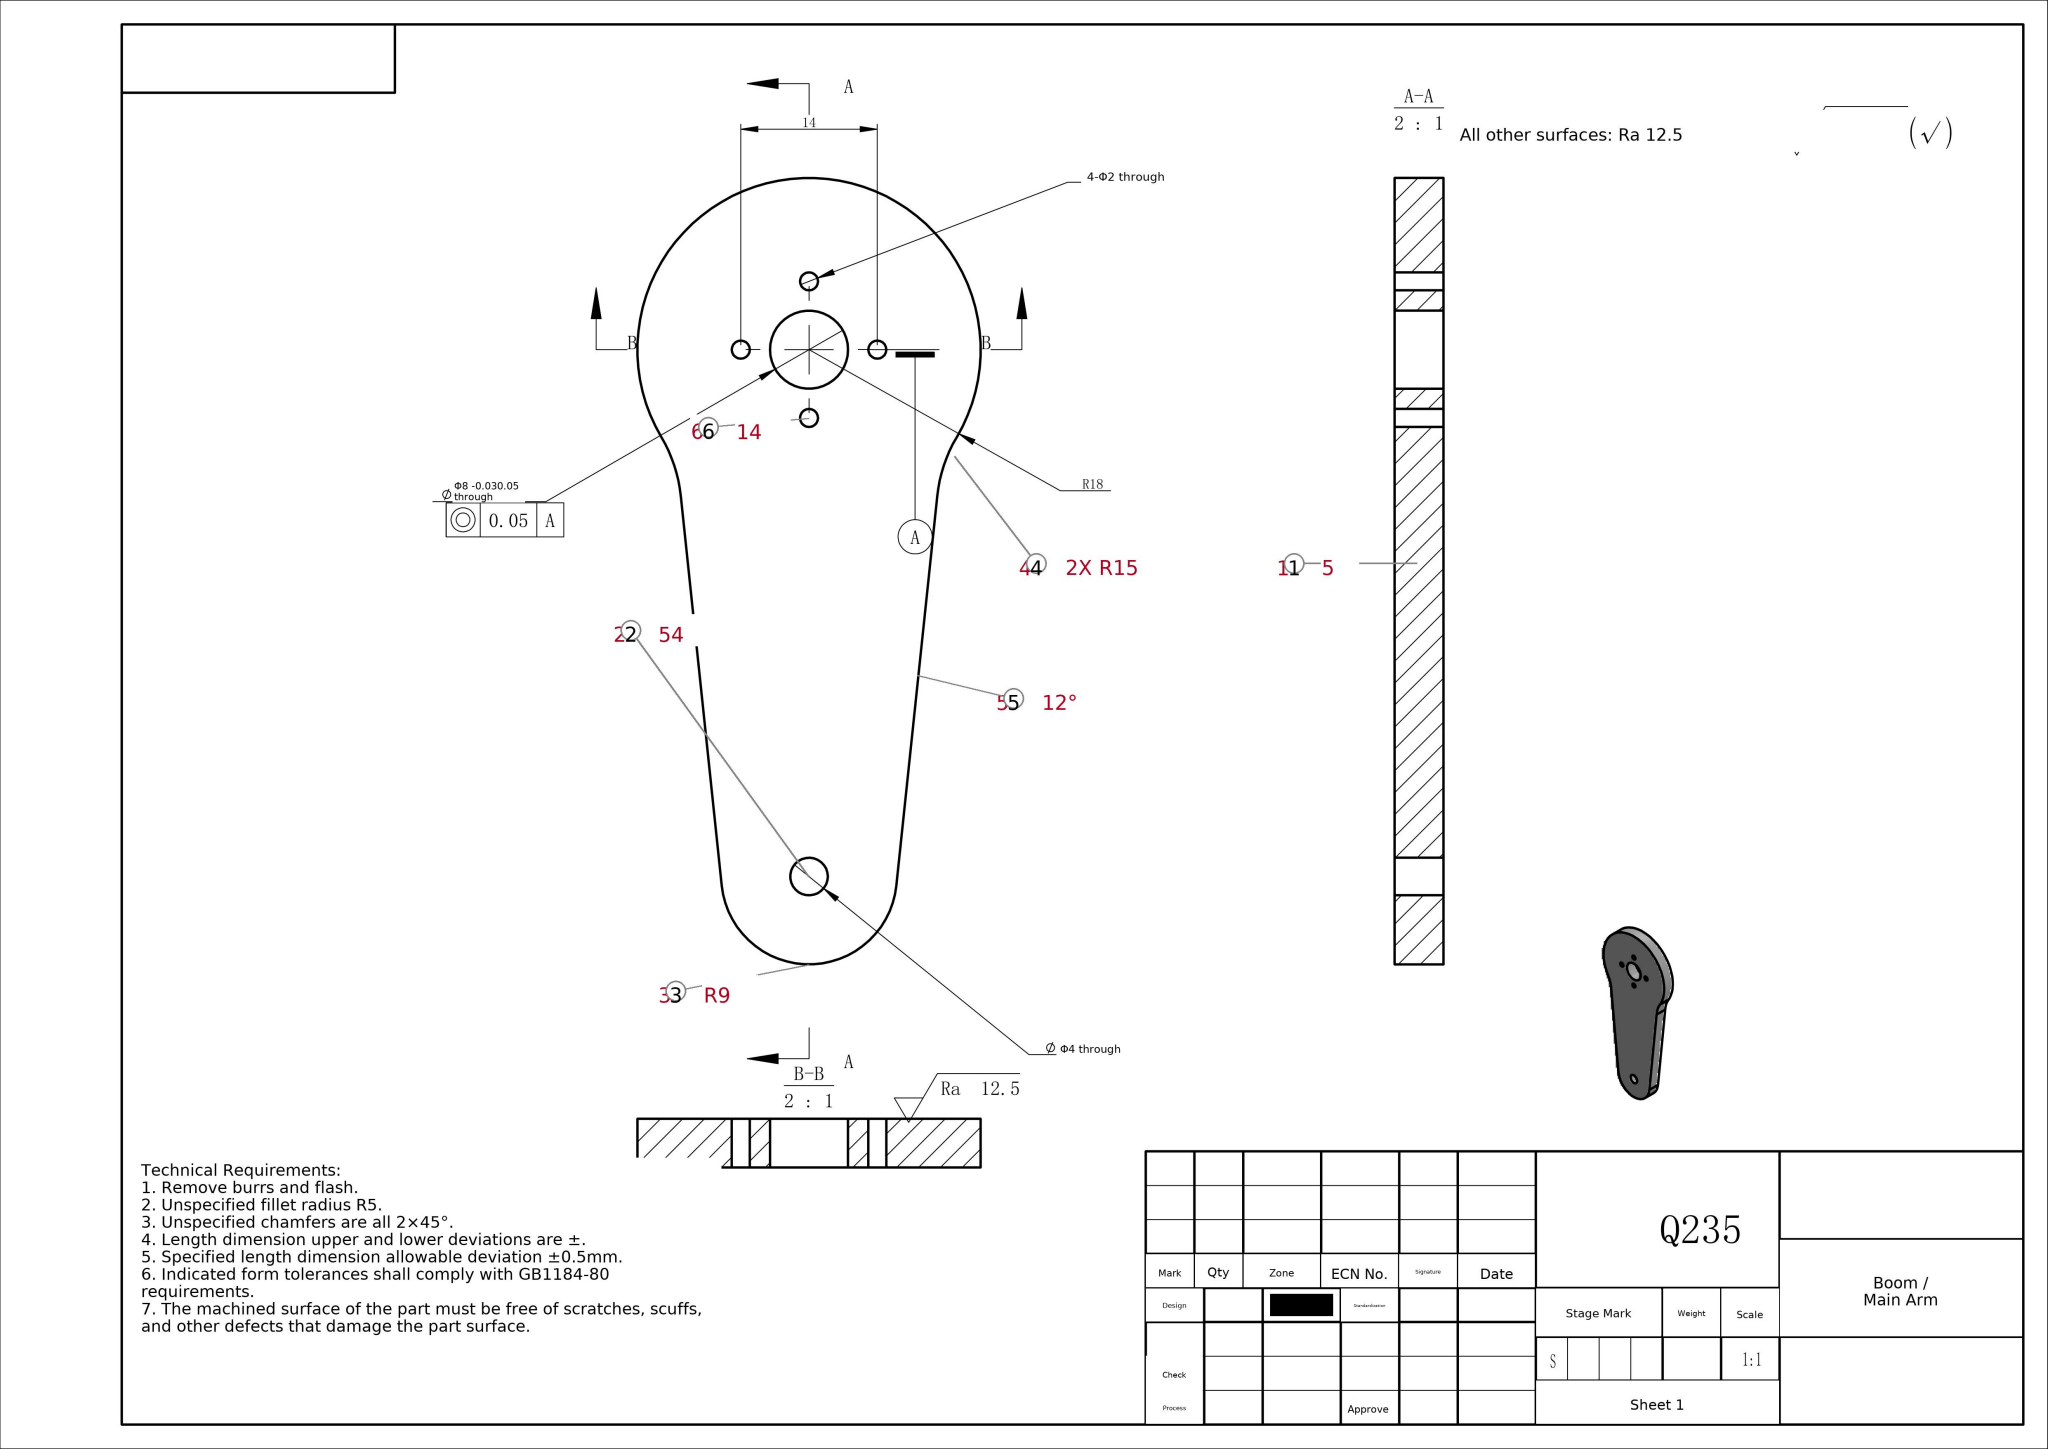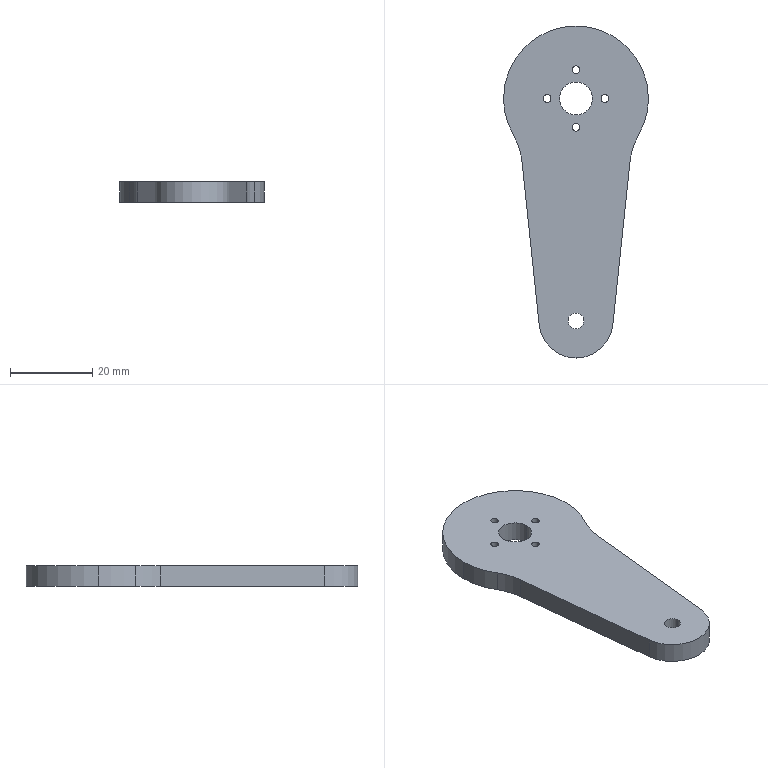Part | SolidWorks | mm | material Q235 | 1 solid | 22 faces | box 35.2 x 80.6 x 5 mm | volume 9381 mm3 | cylinder 18 | plane 4 | commonest cylinder face diameters 1.85 x8 35.2 x3 8 x2 3.85 x2 30 x2 18 x1
build123d program:
from build123d import *

# Parameters (mm, degrees)
ESQUISSE1_R        = 1.925
ESQUISSE1_R_2      = 0.925
ESQUISSE1_R_3      = 4
BOSS_EXTRU_1_DEPTH = 5


with BuildPart() as part:
    # Esquisse1 → Boss.-Extru.1 (new body)
    with BuildSketch(Plane.XY):
        with BuildLine():
            Line((8.951, -54.941), (13.147, -15.02))
            ThreePointArc((13.147, -15.02), (13.822, -11.88), (15.151, -8.955))
            ThreePointArc((15.151, -8.955), (0, 17.6), (-15.151, -8.955))
            ThreePointArc((-15.151, -8.955), (-13.822, -11.88), (-13.147, -15.02))
            Line((-13.147, -15.02), (-8.951, -54.941))
            ThreePointArc((-8.951, -54.941), (0, -63), (8.951, -54.941))
        make_face()
        with Locations((0, -54)):
            Circle(ESQUISSE1_R, mode=Mode.SUBTRACT)
        with Locations((7, 0)):
            Circle(ESQUISSE1_R_2, mode=Mode.SUBTRACT)
        with Locations((0, -7)):
            Circle(ESQUISSE1_R_2, mode=Mode.SUBTRACT)
        with Locations((0, 7)):
            Circle(ESQUISSE1_R_2, mode=Mode.SUBTRACT)
        with Locations((-7, 0)):
            Circle(ESQUISSE1_R_2, mode=Mode.SUBTRACT)
        Circle(ESQUISSE1_R_3, mode=Mode.SUBTRACT)
    extrude(amount=BOSS_EXTRU_1_DEPTH)


solid = part.part
STEP:
#1=CARTESIAN_POINT('',(-4.,0.,5.));
#2=VERTEX_POINT('',#1);
#3=CARTESIAN_POINT('',(4.,0.,5.));
#4=VERTEX_POINT('',#3);
#5=CARTESIAN_POINT('',(0.,0.,5.));
#6=DIRECTION('',(0.,0.,1.));
#7=DIRECTION('',(1.,0.,0.));
#8=AXIS2_PLACEMENT_3D('',#5,#6,#7);
#9=CIRCLE('',#8,4.);
#10=EDGE_CURVE('',#2,#4,#9,.T.);
#11=ORIENTED_EDGE('',*,*,#10,.T.);
#12=CARTESIAN_POINT('',(4.,0.,0.));
#13=VERTEX_POINT('',#12);
#14=CARTESIAN_POINT('',(4.,0.,5.));
#15=DIRECTION('',(0.,0.,-1.));
#16=VECTOR('',#15,1000.);
#17=LINE('',#14,#16);
#18=EDGE_CURVE('',#4,#13,#17,.T.);
#19=ORIENTED_EDGE('',*,*,#18,.T.);
#20=CARTESIAN_POINT('',(-4.,0.,0.));
#21=VERTEX_POINT('',#20);
#22=CARTESIAN_POINT('',(0.,0.,0.));
#23=DIRECTION('',(0.,0.,1.));
#24=DIRECTION('',(1.,0.,0.));
#25=AXIS2_PLACEMENT_3D('',#22,#23,#24);
#26=CIRCLE('',#25,4.);
#27=EDGE_CURVE('',#21,#13,#26,.T.);
#28=ORIENTED_EDGE('',*,*,#27,.F.);
#29=CARTESIAN_POINT('',(-4.,0.,5.));
#30=DIRECTION('',(0.,0.,-1.));
#31=VECTOR('',#30,1000.);
#32=LINE('',#29,#31);
#33=EDGE_CURVE('',#2,#21,#32,.T.);
#34=ORIENTED_EDGE('',*,*,#33,.F.);
#35=EDGE_LOOP('',(#11,#19,#28,#34));
#36=FACE_OUTER_BOUND('',#35,.T.);
#37=CARTESIAN_POINT('',(0.,0.,5.));
#38=DIRECTION('',(0.,0.,-1.));
#39=DIRECTION('',(-1.,0.,0.));
#40=AXIS2_PLACEMENT_3D('',#37,#38,#39);
#41=CYLINDRICAL_SURFACE('',#40,4.);
#42=ADVANCED_FACE('',(#36),#41,.F.);
#43=CARTESIAN_POINT('',(-7.925,0.,5.));
#44=VERTEX_POINT('',#43);
#45=CARTESIAN_POINT('',(-6.075,0.,5.));
#46=VERTEX_POINT('',#45);
#47=CARTESIAN_POINT('',(-7.,0.,5.));
#48=DIRECTION('',(0.,0.,1.));
#49=DIRECTION('',(1.,0.,0.));
#50=AXIS2_PLACEMENT_3D('',#47,#48,#49);
#51=CIRCLE('',#50,0.925);
#52=EDGE_CURVE('',#44,#46,#51,.T.);
#53=ORIENTED_EDGE('',*,*,#52,.T.);
#54=CARTESIAN_POINT('',(-6.075,0.,0.));
#55=VERTEX_POINT('',#54);
#56=CARTESIAN_POINT('',(-6.075,0.,5.));
#57=DIRECTION('',(0.,0.,-1.));
#58=VECTOR('',#57,1000.);
#59=LINE('',#56,#58);
#60=EDGE_CURVE('',#46,#55,#59,.T.);
#61=ORIENTED_EDGE('',*,*,#60,.T.);
#62=CARTESIAN_POINT('',(-7.925,0.,0.));
#63=VERTEX_POINT('',#62);
#64=CARTESIAN_POINT('',(-7.,0.,0.));
#65=DIRECTION('',(0.,0.,1.));
#66=DIRECTION('',(1.,0.,0.));
#67=AXIS2_PLACEMENT_3D('',#64,#65,#66);
#68=CIRCLE('',#67,0.925);
#69=EDGE_CURVE('',#63,#55,#68,.T.);
#70=ORIENTED_EDGE('',*,*,#69,.F.);
#71=CARTESIAN_POINT('',(-7.925,0.,5.));
#72=DIRECTION('',(0.,0.,-1.));
#73=VECTOR('',#72,1000.);
#74=LINE('',#71,#73);
#75=EDGE_CURVE('',#44,#63,#74,.T.);
#76=ORIENTED_EDGE('',*,*,#75,.F.);
#77=EDGE_LOOP('',(#53,#61,#70,#76));
#78=FACE_OUTER_BOUND('',#77,.T.);
#79=CARTESIAN_POINT('',(-7.,0.,5.));
#80=DIRECTION('',(0.,0.,-1.));
#81=DIRECTION('',(-1.,0.,0.));
#82=AXIS2_PLACEMENT_3D('',#79,#80,#81);
#83=CYLINDRICAL_SURFACE('',#82,0.925);
#84=ADVANCED_FACE('',(#78),#83,.F.);
#85=CARTESIAN_POINT('',(-0.925,7.,5.));
#86=VERTEX_POINT('',#85);
#87=CARTESIAN_POINT('',(0.925,7.,5.));
#88=VERTEX_POINT('',#87);
#89=CARTESIAN_POINT('',(0.,7.,5.));
#90=DIRECTION('',(0.,0.,1.));
#91=DIRECTION('',(1.,0.,0.));
#92=AXIS2_PLACEMENT_3D('',#89,#90,#91);
#93=CIRCLE('',#92,0.925);
#94=EDGE_CURVE('',#86,#88,#93,.T.);
#95=ORIENTED_EDGE('',*,*,#94,.T.);
#96=CARTESIAN_POINT('',(0.925,7.,0.));
#97=VERTEX_POINT('',#96);
#98=CARTESIAN_POINT('',(0.925,7.,5.));
#99=DIRECTION('',(0.,0.,-1.));
#100=VECTOR('',#99,1000.);
#101=LINE('',#98,#100);
#102=EDGE_CURVE('',#88,#97,#101,.T.);
#103=ORIENTED_EDGE('',*,*,#102,.T.);
#104=CARTESIAN_POINT('',(-0.925,7.,0.));
#105=VERTEX_POINT('',#104);
#106=CARTESIAN_POINT('',(0.,7.,0.));
#107=DIRECTION('',(0.,0.,1.));
#108=DIRECTION('',(1.,0.,0.));
#109=AXIS2_PLACEMENT_3D('',#106,#107,#108);
#110=CIRCLE('',#109,0.925);
#111=EDGE_CURVE('',#105,#97,#110,.T.);
#112=ORIENTED_EDGE('',*,*,#111,.F.);
#113=CARTESIAN_POINT('',(-0.925,7.,5.));
#114=DIRECTION('',(0.,0.,-1.));
#115=VECTOR('',#114,1000.);
#116=LINE('',#113,#115);
#117=EDGE_CURVE('',#86,#105,#116,.T.);
#118=ORIENTED_EDGE('',*,*,#117,.F.);
#119=EDGE_LOOP('',(#95,#103,#112,#118));
#120=FACE_OUTER_BOUND('',#119,.T.);
#121=CARTESIAN_POINT('',(0.,7.,5.));
#122=DIRECTION('',(0.,0.,-1.));
#123=DIRECTION('',(-1.,0.,0.));
#124=AXIS2_PLACEMENT_3D('',#121,#122,#123);
#125=CYLINDRICAL_SURFACE('',#124,0.925);
#126=ADVANCED_FACE('',(#120),#125,.F.);
#127=CARTESIAN_POINT('',(-0.925,-7.,5.));
#128=VERTEX_POINT('',#127);
#129=CARTESIAN_POINT('',(0.925,-7.,5.));
#130=VERTEX_POINT('',#129);
#131=CARTESIAN_POINT('',(0.,-7.,5.));
#132=DIRECTION('',(0.,0.,1.));
#133=DIRECTION('',(1.,0.,0.));
#134=AXIS2_PLACEMENT_3D('',#131,#132,#133);
#135=CIRCLE('',#134,0.925);
#136=EDGE_CURVE('',#128,#130,#135,.T.);
#137=ORIENTED_EDGE('',*,*,#136,.T.);
#138=CARTESIAN_POINT('',(0.925,-7.,0.));
#139=VERTEX_POINT('',#138);
#140=CARTESIAN_POINT('',(0.925,-7.,5.));
#141=DIRECTION('',(0.,0.,-1.));
#142=VECTOR('',#141,1000.);
#143=LINE('',#140,#142);
#144=EDGE_CURVE('',#130,#139,#143,.T.);
#145=ORIENTED_EDGE('',*,*,#144,.T.);
#146=CARTESIAN_POINT('',(-0.925,-7.,0.));
#147=VERTEX_POINT('',#146);
#148=CARTESIAN_POINT('',(0.,-7.,0.));
#149=DIRECTION('',(0.,0.,1.));
#150=DIRECTION('',(1.,0.,0.));
#151=AXIS2_PLACEMENT_3D('',#148,#149,#150);
#152=CIRCLE('',#151,0.925);
#153=EDGE_CURVE('',#147,#139,#152,.T.);
#154=ORIENTED_EDGE('',*,*,#153,.F.);
#155=CARTESIAN_POINT('',(-0.925,-7.,5.));
#156=DIRECTION('',(0.,0.,-1.));
#157=VECTOR('',#156,1000.);
#158=LINE('',#155,#157);
#159=EDGE_CURVE('',#128,#147,#158,.T.);
#160=ORIENTED_EDGE('',*,*,#159,.F.);
#161=EDGE_LOOP('',(#137,#145,#154,#160));
#162=FACE_OUTER_BOUND('',#161,.T.);
#163=CARTESIAN_POINT('',(0.,-7.,5.));
#164=DIRECTION('',(0.,0.,-1.));
#165=DIRECTION('',(-1.,0.,0.));
#166=AXIS2_PLACEMENT_3D('',#163,#164,#165);
#167=CYLINDRICAL_SURFACE('',#166,0.925);
#168=ADVANCED_FACE('',(#162),#167,.F.);
#169=CARTESIAN_POINT('',(6.075,0.,5.));
#170=VERTEX_POINT('',#169);
#171=CARTESIAN_POINT('',(7.925,0.,5.));
#172=VERTEX_POINT('',#171);
#173=CARTESIAN_POINT('',(7.,0.,5.));
#174=DIRECTION('',(0.,0.,1.));
#175=DIRECTION('',(1.,0.,0.));
#176=AXIS2_PLACEMENT_3D('',#173,#174,#175);
#177=CIRCLE('',#176,0.925);
#178=EDGE_CURVE('',#170,#172,#177,.T.);
#179=ORIENTED_EDGE('',*,*,#178,.T.);
#180=CARTESIAN_POINT('',(7.925,0.,0.));
#181=VERTEX_POINT('',#180);
#182=CARTESIAN_POINT('',(7.925,0.,5.));
#183=DIRECTION('',(0.,0.,-1.));
#184=VECTOR('',#183,1000.);
#185=LINE('',#182,#184);
#186=EDGE_CURVE('',#172,#181,#185,.T.);
#187=ORIENTED_EDGE('',*,*,#186,.T.);
#188=CARTESIAN_POINT('',(6.075,0.,0.));
#189=VERTEX_POINT('',#188);
#190=CARTESIAN_POINT('',(7.,0.,0.));
#191=DIRECTION('',(0.,0.,1.));
#192=DIRECTION('',(1.,0.,0.));
#193=AXIS2_PLACEMENT_3D('',#190,#191,#192);
#194=CIRCLE('',#193,0.925);
#195=EDGE_CURVE('',#189,#181,#194,.T.);
#196=ORIENTED_EDGE('',*,*,#195,.F.);
#197=CARTESIAN_POINT('',(6.075,0.,5.));
#198=DIRECTION('',(0.,0.,-1.));
#199=VECTOR('',#198,1000.);
#200=LINE('',#197,#199);
#201=EDGE_CURVE('',#170,#189,#200,.T.);
#202=ORIENTED_EDGE('',*,*,#201,.F.);
#203=EDGE_LOOP('',(#179,#187,#196,#202));
#204=FACE_OUTER_BOUND('',#203,.T.);
#205=CARTESIAN_POINT('',(7.,0.,5.));
#206=DIRECTION('',(0.,0.,-1.));
#207=DIRECTION('',(-1.,0.,0.));
#208=AXIS2_PLACEMENT_3D('',#205,#206,#207);
#209=CYLINDRICAL_SURFACE('',#208,0.925);
#210=ADVANCED_FACE('',(#204),#209,.F.);
#211=CARTESIAN_POINT('',(-1.925,-54.,5.));
#212=VERTEX_POINT('',#211);
#213=CARTESIAN_POINT('',(1.925,-54.,5.));
#214=VERTEX_POINT('',#213);
#215=CARTESIAN_POINT('',(0.,-54.,5.));
#216=DIRECTION('',(0.,0.,1.));
#217=DIRECTION('',(1.,0.,0.));
#218=AXIS2_PLACEMENT_3D('',#215,#216,#217);
#219=CIRCLE('',#218,1.925);
#220=EDGE_CURVE('',#212,#214,#219,.T.);
#221=ORIENTED_EDGE('',*,*,#220,.T.);
#222=CARTESIAN_POINT('',(1.925,-54.,0.));
#223=VERTEX_POINT('',#222);
#224=CARTESIAN_POINT('',(1.925,-54.,5.));
#225=DIRECTION('',(0.,0.,-1.));
#226=VECTOR('',#225,1000.);
#227=LINE('',#224,#226);
#228=EDGE_CURVE('',#214,#223,#227,.T.);
#229=ORIENTED_EDGE('',*,*,#228,.T.);
#230=CARTESIAN_POINT('',(-1.925,-54.,0.));
#231=VERTEX_POINT('',#230);
#232=CARTESIAN_POINT('',(0.,-54.,0.));
#233=DIRECTION('',(0.,0.,1.));
#234=DIRECTION('',(1.,0.,0.));
#235=AXIS2_PLACEMENT_3D('',#232,#233,#234);
#236=CIRCLE('',#235,1.925);
#237=EDGE_CURVE('',#231,#223,#236,.T.);
#238=ORIENTED_EDGE('',*,*,#237,.F.);
#239=CARTESIAN_POINT('',(-1.925,-54.,5.));
#240=DIRECTION('',(0.,0.,-1.));
#241=VECTOR('',#240,1000.);
#242=LINE('',#239,#241);
#243=EDGE_CURVE('',#212,#231,#242,.T.);
#244=ORIENTED_EDGE('',*,*,#243,.F.);
#245=EDGE_LOOP('',(#221,#229,#238,#244));
#246=FACE_OUTER_BOUND('',#245,.T.);
#247=CARTESIAN_POINT('',(0.,-54.,5.));
#248=DIRECTION('',(0.,0.,-1.));
#249=DIRECTION('',(-1.,0.,0.));
#250=AXIS2_PLACEMENT_3D('',#247,#248,#249);
#251=CYLINDRICAL_SURFACE('',#250,1.925);
#252=ADVANCED_FACE('',(#246),#251,.F.);
#253=CARTESIAN_POINT('',(17.6,0.,5.));
#254=VERTEX_POINT('',#253);
#255=CARTESIAN_POINT('',(-17.6,0.,5.));
#256=VERTEX_POINT('',#255);
#257=CARTESIAN_POINT('',(0.,0.,5.));
#258=DIRECTION('',(0.,0.,1.));
#259=DIRECTION('',(1.,0.,0.));
#260=AXIS2_PLACEMENT_3D('',#257,#258,#259);
#261=CIRCLE('',#260,17.6);
#262=EDGE_CURVE('',#254,#256,#261,.T.);
#263=ORIENTED_EDGE('',*,*,#262,.F.);
#264=CARTESIAN_POINT('',(17.6,0.,0.));
#265=VERTEX_POINT('',#264);
#266=CARTESIAN_POINT('',(17.6,0.,5.));
#267=DIRECTION('',(0.,0.,-1.));
#268=VECTOR('',#267,1000.);
#269=LINE('',#266,#268);
#270=EDGE_CURVE('',#254,#265,#269,.T.);
#271=ORIENTED_EDGE('',*,*,#270,.T.);
#272=CARTESIAN_POINT('',(-17.6,0.,0.));
#273=VERTEX_POINT('',#272);
#274=CARTESIAN_POINT('',(0.,0.,0.));
#275=DIRECTION('',(0.,0.,1.));
#276=DIRECTION('',(1.,0.,0.));
#277=AXIS2_PLACEMENT_3D('',#274,#275,#276);
#278=CIRCLE('',#277,17.6);
#279=EDGE_CURVE('',#265,#273,#278,.T.);
#280=ORIENTED_EDGE('',*,*,#279,.T.);
#281=CARTESIAN_POINT('',(-17.6,0.,5.));
#282=DIRECTION('',(0.,0.,-1.));
#283=VECTOR('',#282,1000.);
#284=LINE('',#281,#283);
#285=EDGE_CURVE('',#256,#273,#284,.T.);
#286=ORIENTED_EDGE('',*,*,#285,.F.);
#287=EDGE_LOOP('',(#263,#271,#280,#286));
#288=FACE_OUTER_BOUND('',#287,.T.);
#289=CARTESIAN_POINT('',(0.,0.,5.));
#290=DIRECTION('',(0.,0.,-1.));
#291=DIRECTION('',(-1.,0.,0.));
#292=AXIS2_PLACEMENT_3D('',#289,#290,#291);
#293=CYLINDRICAL_SURFACE('',#292,17.6);
#294=ADVANCED_FACE('',(#288),#293,.T.);
#295=CARTESIAN_POINT('',(-15.151,-8.955,5.));
#296=VERTEX_POINT('',#295);
#297=CARTESIAN_POINT('',(0.,0.,5.));
#298=DIRECTION('',(0.,0.,1.));
#299=DIRECTION('',(1.,0.,0.));
#300=AXIS2_PLACEMENT_3D('',#297,#298,#299);
#301=CIRCLE('',#300,17.6);
#302=EDGE_CURVE('',#256,#296,#301,.T.);
#303=ORIENTED_EDGE('',*,*,#302,.F.);
#304=ORIENTED_EDGE('',*,*,#285,.T.);
#305=CARTESIAN_POINT('',(-15.151,-8.955,0.));
#306=VERTEX_POINT('',#305);
#307=CARTESIAN_POINT('',(0.,0.,0.));
#308=DIRECTION('',(0.,0.,1.));
#309=DIRECTION('',(1.,0.,0.));
#310=AXIS2_PLACEMENT_3D('',#307,#308,#309);
#311=CIRCLE('',#310,17.6);
#312=EDGE_CURVE('',#273,#306,#311,.T.);
#313=ORIENTED_EDGE('',*,*,#312,.T.);
#314=CARTESIAN_POINT('',(-15.151,-8.955,5.));
#315=DIRECTION('',(0.,0.,-1.));
#316=VECTOR('',#315,1000.);
#317=LINE('',#314,#316);
#318=EDGE_CURVE('',#296,#306,#317,.T.);
#319=ORIENTED_EDGE('',*,*,#318,.F.);
#320=EDGE_LOOP('',(#303,#304,#313,#319));
#321=FACE_OUTER_BOUND('',#320,.T.);
#322=CARTESIAN_POINT('',(0.,0.,5.));
#323=DIRECTION('',(0.,0.,-1.));
#324=DIRECTION('',(-1.,0.,0.));
#325=AXIS2_PLACEMENT_3D('',#322,#323,#324);
#326=CYLINDRICAL_SURFACE('',#325,17.6);
#327=ADVANCED_FACE('',(#321),#326,.T.);
#328=ORIENTED_EDGE('',*,*,#52,.F.);
#329=CARTESIAN_POINT('',(-7.,0.,5.));
#330=DIRECTION('',(0.,0.,1.));
#331=DIRECTION('',(1.,0.,0.));
#332=AXIS2_PLACEMENT_3D('',#329,#330,#331);
#333=CIRCLE('',#332,0.925);
#334=EDGE_CURVE('',#46,#44,#333,.T.);
#335=ORIENTED_EDGE('',*,*,#334,.F.);
#336=EDGE_LOOP('',(#328,#335));
#337=FACE_BOUND('',#336,.T.);
#338=ORIENTED_EDGE('',*,*,#136,.F.);
#339=CARTESIAN_POINT('',(0.,-7.,5.));
#340=DIRECTION('',(0.,0.,1.));
#341=DIRECTION('',(1.,0.,0.));
#342=AXIS2_PLACEMENT_3D('',#339,#340,#341);
#343=CIRCLE('',#342,0.925);
#344=EDGE_CURVE('',#130,#128,#343,.T.);
#345=ORIENTED_EDGE('',*,*,#344,.F.);
#346=EDGE_LOOP('',(#338,#345));
#347=FACE_BOUND('',#346,.T.);
#348=ORIENTED_EDGE('',*,*,#220,.F.);
#349=CARTESIAN_POINT('',(0.,-54.,5.));
#350=DIRECTION('',(0.,0.,1.));
#351=DIRECTION('',(1.,0.,0.));
#352=AXIS2_PLACEMENT_3D('',#349,#350,#351);
#353=CIRCLE('',#352,1.925);
#354=EDGE_CURVE('',#214,#212,#353,.T.);
#355=ORIENTED_EDGE('',*,*,#354,.F.);
#356=EDGE_LOOP('',(#348,#355));
#357=FACE_BOUND('',#356,.T.);
#358=CARTESIAN_POINT('',(-8.951,-54.941,5.));
#359=VERTEX_POINT('',#358);
#360=CARTESIAN_POINT('',(8.951,-54.941,5.));
#361=VERTEX_POINT('',#360);
#362=CARTESIAN_POINT('',(0.,-54.,5.));
#363=DIRECTION('',(0.,0.,1.));
#364=DIRECTION('',(1.,0.,0.));
#365=AXIS2_PLACEMENT_3D('',#362,#363,#364);
#366=CIRCLE('',#365,9.);
#367=EDGE_CURVE('',#359,#361,#366,.T.);
#368=ORIENTED_EDGE('',*,*,#367,.T.);
#369=CARTESIAN_POINT('',(13.147,-15.02,5.));
#370=VERTEX_POINT('',#369);
#371=CARTESIAN_POINT('',(8.951,-54.941,5.));
#372=DIRECTION('',(0.1045,0.9945,0.));
#373=VECTOR('',#372,1000.);
#374=LINE('',#371,#373);
#375=EDGE_CURVE('',#361,#370,#374,.T.);
#376=ORIENTED_EDGE('',*,*,#375,.T.);
#377=CARTESIAN_POINT('',(15.151,-8.955,5.));
#378=VERTEX_POINT('',#377);
#379=CARTESIAN_POINT('',(28.064,-16.588,5.));
#380=DIRECTION('',(0.,0.,-1.));
#381=DIRECTION('',(1.,0.,0.));
#382=AXIS2_PLACEMENT_3D('',#379,#380,#381);
#383=CIRCLE('',#382,15.);
#384=EDGE_CURVE('',#370,#378,#383,.T.);
#385=ORIENTED_EDGE('',*,*,#384,.T.);
#386=CARTESIAN_POINT('',(0.,0.,5.));
#387=DIRECTION('',(0.,0.,1.));
#388=DIRECTION('',(1.,0.,0.));
#389=AXIS2_PLACEMENT_3D('',#386,#387,#388);
#390=CIRCLE('',#389,17.6);
#391=EDGE_CURVE('',#378,#254,#390,.T.);
#392=ORIENTED_EDGE('',*,*,#391,.T.);
#393=ORIENTED_EDGE('',*,*,#262,.T.);
#394=ORIENTED_EDGE('',*,*,#302,.T.);
#395=CARTESIAN_POINT('',(-13.147,-15.02,5.));
#396=VERTEX_POINT('',#395);
#397=CARTESIAN_POINT('',(-28.064,-16.588,5.));
#398=DIRECTION('',(0.,0.,-1.));
#399=DIRECTION('',(1.,0.,0.));
#400=AXIS2_PLACEMENT_3D('',#397,#398,#399);
#401=CIRCLE('',#400,15.);
#402=EDGE_CURVE('',#296,#396,#401,.T.);
#403=ORIENTED_EDGE('',*,*,#402,.T.);
#404=CARTESIAN_POINT('',(-13.147,-15.02,5.));
#405=DIRECTION('',(0.1045,-0.9945,0.));
#406=VECTOR('',#405,1000.);
#407=LINE('',#404,#406);
#408=EDGE_CURVE('',#396,#359,#407,.T.);
#409=ORIENTED_EDGE('',*,*,#408,.T.);
#410=EDGE_LOOP('',(#368,#376,#385,#392,#393,#394,#403,#409));
#411=FACE_OUTER_BOUND('',#410,.T.);
#412=ORIENTED_EDGE('',*,*,#178,.F.);
#413=CARTESIAN_POINT('',(7.,0.,5.));
#414=DIRECTION('',(0.,0.,1.));
#415=DIRECTION('',(1.,0.,0.));
#416=AXIS2_PLACEMENT_3D('',#413,#414,#415);
#417=CIRCLE('',#416,0.925);
#418=EDGE_CURVE('',#172,#170,#417,.T.);
#419=ORIENTED_EDGE('',*,*,#418,.F.);
#420=EDGE_LOOP('',(#412,#419));
#421=FACE_BOUND('',#420,.T.);
#422=ORIENTED_EDGE('',*,*,#94,.F.);
#423=CARTESIAN_POINT('',(0.,7.,5.));
#424=DIRECTION('',(0.,0.,1.));
#425=DIRECTION('',(1.,0.,0.));
#426=AXIS2_PLACEMENT_3D('',#423,#424,#425);
#427=CIRCLE('',#426,0.925);
#428=EDGE_CURVE('',#88,#86,#427,.T.);
#429=ORIENTED_EDGE('',*,*,#428,.F.);
#430=EDGE_LOOP('',(#422,#429));
#431=FACE_BOUND('',#430,.T.);
#432=ORIENTED_EDGE('',*,*,#10,.F.);
#433=CARTESIAN_POINT('',(0.,0.,5.));
#434=DIRECTION('',(0.,0.,1.));
#435=DIRECTION('',(1.,0.,0.));
#436=AXIS2_PLACEMENT_3D('',#433,#434,#435);
#437=CIRCLE('',#436,4.);
#438=EDGE_CURVE('',#4,#2,#437,.T.);
#439=ORIENTED_EDGE('',*,*,#438,.F.);
#440=EDGE_LOOP('',(#432,#439));
#441=FACE_BOUND('',#440,.T.);
#442=CARTESIAN_POINT('',(0.,-54.,5.));
#443=DIRECTION('',(0.,0.,1.));
#444=DIRECTION('',(1.,0.,0.));
#445=AXIS2_PLACEMENT_3D('',#442,#443,#444);
#446=PLANE('',#445);
#447=ADVANCED_FACE('',(#337,#347,#357,#411,#421,#431,#441),#446,.T.);
#448=CARTESIAN_POINT('',(-8.951,-54.941,0.));
#449=VERTEX_POINT('',#448);
#450=CARTESIAN_POINT('',(8.951,-54.941,0.));
#451=VERTEX_POINT('',#450);
#452=CARTESIAN_POINT('',(0.,-54.,0.));
#453=DIRECTION('',(0.,0.,1.));
#454=DIRECTION('',(1.,0.,0.));
#455=AXIS2_PLACEMENT_3D('',#452,#453,#454);
#456=CIRCLE('',#455,9.);
#457=EDGE_CURVE('',#449,#451,#456,.T.);
#458=ORIENTED_EDGE('',*,*,#457,.F.);
#459=CARTESIAN_POINT('',(-13.147,-15.02,0.));
#460=VERTEX_POINT('',#459);
#461=CARTESIAN_POINT('',(-13.147,-15.02,0.));
#462=DIRECTION('',(0.1045,-0.9945,0.));
#463=VECTOR('',#462,1000.);
#464=LINE('',#461,#463);
#465=EDGE_CURVE('',#460,#449,#464,.T.);
#466=ORIENTED_EDGE('',*,*,#465,.F.);
#467=CARTESIAN_POINT('',(-28.064,-16.588,0.));
#468=DIRECTION('',(0.,0.,-1.));
#469=DIRECTION('',(1.,0.,0.));
#470=AXIS2_PLACEMENT_3D('',#467,#468,#469);
#471=CIRCLE('',#470,15.);
#472=EDGE_CURVE('',#306,#460,#471,.T.);
#473=ORIENTED_EDGE('',*,*,#472,.F.);
#474=ORIENTED_EDGE('',*,*,#312,.F.);
#475=ORIENTED_EDGE('',*,*,#279,.F.);
#476=CARTESIAN_POINT('',(15.151,-8.955,0.));
#477=VERTEX_POINT('',#476);
#478=CARTESIAN_POINT('',(0.,0.,0.));
#479=DIRECTION('',(0.,0.,1.));
#480=DIRECTION('',(1.,0.,0.));
#481=AXIS2_PLACEMENT_3D('',#478,#479,#480);
#482=CIRCLE('',#481,17.6);
#483=EDGE_CURVE('',#477,#265,#482,.T.);
#484=ORIENTED_EDGE('',*,*,#483,.F.);
#485=CARTESIAN_POINT('',(13.147,-15.02,0.));
#486=VERTEX_POINT('',#485);
#487=CARTESIAN_POINT('',(28.064,-16.588,0.));
#488=DIRECTION('',(0.,0.,-1.));
#489=DIRECTION('',(1.,0.,0.));
#490=AXIS2_PLACEMENT_3D('',#487,#488,#489);
#491=CIRCLE('',#490,15.);
#492=EDGE_CURVE('',#486,#477,#491,.T.);
#493=ORIENTED_EDGE('',*,*,#492,.F.);
#494=CARTESIAN_POINT('',(8.951,-54.941,0.));
#495=DIRECTION('',(0.1045,0.9945,0.));
#496=VECTOR('',#495,1000.);
#497=LINE('',#494,#496);
#498=EDGE_CURVE('',#451,#486,#497,.T.);
#499=ORIENTED_EDGE('',*,*,#498,.F.);
#500=EDGE_LOOP('',(#458,#466,#473,#474,#475,#484,#493,#499));
#501=FACE_OUTER_BOUND('',#500,.T.);
#502=ORIENTED_EDGE('',*,*,#237,.T.);
#503=CARTESIAN_POINT('',(0.,-54.,0.));
#504=DIRECTION('',(0.,0.,1.));
#505=DIRECTION('',(1.,0.,0.));
#506=AXIS2_PLACEMENT_3D('',#503,#504,#505);
#507=CIRCLE('',#506,1.925);
#508=EDGE_CURVE('',#223,#231,#507,.T.);
#509=ORIENTED_EDGE('',*,*,#508,.T.);
#510=EDGE_LOOP('',(#502,#509));
#511=FACE_BOUND('',#510,.T.);
#512=ORIENTED_EDGE('',*,*,#195,.T.);
#513=CARTESIAN_POINT('',(7.,0.,0.));
#514=DIRECTION('',(0.,0.,1.));
#515=DIRECTION('',(1.,0.,0.));
#516=AXIS2_PLACEMENT_3D('',#513,#514,#515);
#517=CIRCLE('',#516,0.925);
#518=EDGE_CURVE('',#181,#189,#517,.T.);
#519=ORIENTED_EDGE('',*,*,#518,.T.);
#520=EDGE_LOOP('',(#512,#519));
#521=FACE_BOUND('',#520,.T.);
#522=ORIENTED_EDGE('',*,*,#153,.T.);
#523=CARTESIAN_POINT('',(0.,-7.,0.));
#524=DIRECTION('',(0.,0.,1.));
#525=DIRECTION('',(1.,0.,0.));
#526=AXIS2_PLACEMENT_3D('',#523,#524,#525);
#527=CIRCLE('',#526,0.925);
#528=EDGE_CURVE('',#139,#147,#527,.T.);
#529=ORIENTED_EDGE('',*,*,#528,.T.);
#530=EDGE_LOOP('',(#522,#529));
#531=FACE_BOUND('',#530,.T.);
#532=ORIENTED_EDGE('',*,*,#111,.T.);
#533=CARTESIAN_POINT('',(0.,7.,0.));
#534=DIRECTION('',(0.,0.,1.));
#535=DIRECTION('',(1.,0.,0.));
#536=AXIS2_PLACEMENT_3D('',#533,#534,#535);
#537=CIRCLE('',#536,0.925);
#538=EDGE_CURVE('',#97,#105,#537,.T.);
#539=ORIENTED_EDGE('',*,*,#538,.T.);
#540=EDGE_LOOP('',(#532,#539));
#541=FACE_BOUND('',#540,.T.);
#542=ORIENTED_EDGE('',*,*,#69,.T.);
#543=CARTESIAN_POINT('',(-7.,0.,0.));
#544=DIRECTION('',(0.,0.,1.));
#545=DIRECTION('',(1.,0.,0.));
#546=AXIS2_PLACEMENT_3D('',#543,#544,#545);
#547=CIRCLE('',#546,0.925);
#548=EDGE_CURVE('',#55,#63,#547,.T.);
#549=ORIENTED_EDGE('',*,*,#548,.T.);
#550=EDGE_LOOP('',(#542,#549));
#551=FACE_BOUND('',#550,.T.);
#552=ORIENTED_EDGE('',*,*,#27,.T.);
#553=CARTESIAN_POINT('',(0.,0.,0.));
#554=DIRECTION('',(0.,0.,1.));
#555=DIRECTION('',(1.,0.,0.));
#556=AXIS2_PLACEMENT_3D('',#553,#554,#555);
#557=CIRCLE('',#556,4.);
#558=EDGE_CURVE('',#13,#21,#557,.T.);
#559=ORIENTED_EDGE('',*,*,#558,.T.);
#560=EDGE_LOOP('',(#552,#559));
#561=FACE_BOUND('',#560,.T.);
#562=CARTESIAN_POINT('',(0.,-54.,0.));
#563=DIRECTION('',(0.,0.,1.));
#564=DIRECTION('',(1.,0.,0.));
#565=AXIS2_PLACEMENT_3D('',#562,#563,#564);
#566=PLANE('',#565);
#567=ADVANCED_FACE('',(#501,#511,#521,#531,#541,#551,#561),#566,.F.);
#568=ORIENTED_EDGE('',*,*,#457,.T.);
#569=CARTESIAN_POINT('',(8.951,-54.941,5.));
#570=DIRECTION('',(0.,0.,-1.));
#571=VECTOR('',#570,1000.);
#572=LINE('',#569,#571);
#573=EDGE_CURVE('',#361,#451,#572,.T.);
#574=ORIENTED_EDGE('',*,*,#573,.F.);
#575=ORIENTED_EDGE('',*,*,#367,.F.);
#576=CARTESIAN_POINT('',(-8.951,-54.941,5.));
#577=DIRECTION('',(0.,0.,-1.));
#578=VECTOR('',#577,1000.);
#579=LINE('',#576,#578);
#580=EDGE_CURVE('',#359,#449,#579,.T.);
#581=ORIENTED_EDGE('',*,*,#580,.T.);
#582=EDGE_LOOP('',(#568,#574,#575,#581));
#583=FACE_OUTER_BOUND('',#582,.T.);
#584=CARTESIAN_POINT('',(0.,-54.,5.));
#585=DIRECTION('',(0.,0.,-1.));
#586=DIRECTION('',(-1.,0.,0.));
#587=AXIS2_PLACEMENT_3D('',#584,#585,#586);
#588=CYLINDRICAL_SURFACE('',#587,9.);
#589=ADVANCED_FACE('',(#583),#588,.T.);
#590=ORIENTED_EDGE('',*,*,#498,.T.);
#591=CARTESIAN_POINT('',(13.147,-15.02,5.));
#592=DIRECTION('',(0.,0.,-1.));
#593=VECTOR('',#592,1000.);
#594=LINE('',#591,#593);
#595=EDGE_CURVE('',#370,#486,#594,.T.);
#596=ORIENTED_EDGE('',*,*,#595,.F.);
#597=ORIENTED_EDGE('',*,*,#375,.F.);
#598=ORIENTED_EDGE('',*,*,#573,.T.);
#599=EDGE_LOOP('',(#590,#596,#597,#598));
#600=FACE_OUTER_BOUND('',#599,.T.);
#601=CARTESIAN_POINT('',(8.951,-54.941,5.));
#602=DIRECTION('',(-0.9945,0.1045,0.));
#603=DIRECTION('',(-0.1045,-0.9945,0.));
#604=AXIS2_PLACEMENT_3D('',#601,#602,#603);
#605=PLANE('',#604);
#606=ADVANCED_FACE('',(#600),#605,.F.);
#607=ORIENTED_EDGE('',*,*,#492,.T.);
#608=CARTESIAN_POINT('',(15.151,-8.955,5.));
#609=DIRECTION('',(0.,0.,-1.));
#610=VECTOR('',#609,1000.);
#611=LINE('',#608,#610);
#612=EDGE_CURVE('',#378,#477,#611,.T.);
#613=ORIENTED_EDGE('',*,*,#612,.F.);
#614=ORIENTED_EDGE('',*,*,#384,.F.);
#615=ORIENTED_EDGE('',*,*,#595,.T.);
#616=EDGE_LOOP('',(#607,#613,#614,#615));
#617=FACE_OUTER_BOUND('',#616,.T.);
#618=CARTESIAN_POINT('',(28.064,-16.588,5.));
#619=DIRECTION('',(0.,0.,-1.));
#620=DIRECTION('',(-1.,0.,0.));
#621=AXIS2_PLACEMENT_3D('',#618,#619,#620);
#622=CYLINDRICAL_SURFACE('',#621,15.);
#623=ADVANCED_FACE('',(#617),#622,.F.);
#624=ORIENTED_EDGE('',*,*,#270,.F.);
#625=ORIENTED_EDGE('',*,*,#391,.F.);
#626=ORIENTED_EDGE('',*,*,#612,.T.);
#627=ORIENTED_EDGE('',*,*,#483,.T.);
#628=EDGE_LOOP('',(#624,#625,#626,#627));
#629=FACE_OUTER_BOUND('',#628,.T.);
#630=CARTESIAN_POINT('',(0.,0.,5.));
#631=DIRECTION('',(0.,0.,-1.));
#632=DIRECTION('',(-1.,0.,0.));
#633=AXIS2_PLACEMENT_3D('',#630,#631,#632);
#634=CYLINDRICAL_SURFACE('',#633,17.6);
#635=ADVANCED_FACE('',(#629),#634,.T.);
#636=ORIENTED_EDGE('',*,*,#472,.T.);
#637=CARTESIAN_POINT('',(-13.147,-15.02,5.));
#638=DIRECTION('',(0.,0.,-1.));
#639=VECTOR('',#638,1000.);
#640=LINE('',#637,#639);
#641=EDGE_CURVE('',#396,#460,#640,.T.);
#642=ORIENTED_EDGE('',*,*,#641,.F.);
#643=ORIENTED_EDGE('',*,*,#402,.F.);
#644=ORIENTED_EDGE('',*,*,#318,.T.);
#645=EDGE_LOOP('',(#636,#642,#643,#644));
#646=FACE_OUTER_BOUND('',#645,.T.);
#647=CARTESIAN_POINT('',(-28.064,-16.588,5.));
#648=DIRECTION('',(0.,0.,-1.));
#649=DIRECTION('',(-1.,0.,0.));
#650=AXIS2_PLACEMENT_3D('',#647,#648,#649);
#651=CYLINDRICAL_SURFACE('',#650,15.);
#652=ADVANCED_FACE('',(#646),#651,.F.);
#653=ORIENTED_EDGE('',*,*,#465,.T.);
#654=ORIENTED_EDGE('',*,*,#580,.F.);
#655=ORIENTED_EDGE('',*,*,#408,.F.);
#656=ORIENTED_EDGE('',*,*,#641,.T.);
#657=EDGE_LOOP('',(#653,#654,#655,#656));
#658=FACE_OUTER_BOUND('',#657,.T.);
#659=CARTESIAN_POINT('',(-13.147,-15.02,5.));
#660=DIRECTION('',(0.9945,0.1045,0.));
#661=DIRECTION('',(-0.1045,0.9945,0.));
#662=AXIS2_PLACEMENT_3D('',#659,#660,#661);
#663=PLANE('',#662);
#664=ADVANCED_FACE('',(#658),#663,.F.);
#665=ORIENTED_EDGE('',*,*,#228,.F.);
#666=ORIENTED_EDGE('',*,*,#354,.T.);
#667=ORIENTED_EDGE('',*,*,#243,.T.);
#668=ORIENTED_EDGE('',*,*,#508,.F.);
#669=EDGE_LOOP('',(#665,#666,#667,#668));
#670=FACE_OUTER_BOUND('',#669,.T.);
#671=CARTESIAN_POINT('',(0.,-54.,5.));
#672=DIRECTION('',(0.,0.,-1.));
#673=DIRECTION('',(-1.,0.,0.));
#674=AXIS2_PLACEMENT_3D('',#671,#672,#673);
#675=CYLINDRICAL_SURFACE('',#674,1.925);
#676=ADVANCED_FACE('',(#670),#675,.F.);
#677=ORIENTED_EDGE('',*,*,#186,.F.);
#678=ORIENTED_EDGE('',*,*,#418,.T.);
#679=ORIENTED_EDGE('',*,*,#201,.T.);
#680=ORIENTED_EDGE('',*,*,#518,.F.);
#681=EDGE_LOOP('',(#677,#678,#679,#680));
#682=FACE_OUTER_BOUND('',#681,.T.);
#683=CARTESIAN_POINT('',(7.,0.,5.));
#684=DIRECTION('',(0.,0.,-1.));
#685=DIRECTION('',(-1.,0.,0.));
#686=AXIS2_PLACEMENT_3D('',#683,#684,#685);
#687=CYLINDRICAL_SURFACE('',#686,0.925);
#688=ADVANCED_FACE('',(#682),#687,.F.);
#689=ORIENTED_EDGE('',*,*,#144,.F.);
#690=ORIENTED_EDGE('',*,*,#344,.T.);
#691=ORIENTED_EDGE('',*,*,#159,.T.);
#692=ORIENTED_EDGE('',*,*,#528,.F.);
#693=EDGE_LOOP('',(#689,#690,#691,#692));
#694=FACE_OUTER_BOUND('',#693,.T.);
#695=CARTESIAN_POINT('',(0.,-7.,5.));
#696=DIRECTION('',(0.,0.,-1.));
#697=DIRECTION('',(-1.,0.,0.));
#698=AXIS2_PLACEMENT_3D('',#695,#696,#697);
#699=CYLINDRICAL_SURFACE('',#698,0.925);
#700=ADVANCED_FACE('',(#694),#699,.F.);
#701=ORIENTED_EDGE('',*,*,#102,.F.);
#702=ORIENTED_EDGE('',*,*,#428,.T.);
#703=ORIENTED_EDGE('',*,*,#117,.T.);
#704=ORIENTED_EDGE('',*,*,#538,.F.);
#705=EDGE_LOOP('',(#701,#702,#703,#704));
#706=FACE_OUTER_BOUND('',#705,.T.);
#707=CARTESIAN_POINT('',(0.,7.,5.));
#708=DIRECTION('',(0.,0.,-1.));
#709=DIRECTION('',(-1.,0.,0.));
#710=AXIS2_PLACEMENT_3D('',#707,#708,#709);
#711=CYLINDRICAL_SURFACE('',#710,0.925);
#712=ADVANCED_FACE('',(#706),#711,.F.);
#713=ORIENTED_EDGE('',*,*,#60,.F.);
#714=ORIENTED_EDGE('',*,*,#334,.T.);
#715=ORIENTED_EDGE('',*,*,#75,.T.);
#716=ORIENTED_EDGE('',*,*,#548,.F.);
#717=EDGE_LOOP('',(#713,#714,#715,#716));
#718=FACE_OUTER_BOUND('',#717,.T.);
#719=CARTESIAN_POINT('',(-7.,0.,5.));
#720=DIRECTION('',(0.,0.,-1.));
#721=DIRECTION('',(-1.,0.,0.));
#722=AXIS2_PLACEMENT_3D('',#719,#720,#721);
#723=CYLINDRICAL_SURFACE('',#722,0.925);
#724=ADVANCED_FACE('',(#718),#723,.F.);
#725=ORIENTED_EDGE('',*,*,#18,.F.);
#726=ORIENTED_EDGE('',*,*,#438,.T.);
#727=ORIENTED_EDGE('',*,*,#33,.T.);
#728=ORIENTED_EDGE('',*,*,#558,.F.);
#729=EDGE_LOOP('',(#725,#726,#727,#728));
#730=FACE_OUTER_BOUND('',#729,.T.);
#731=CARTESIAN_POINT('',(0.,0.,5.));
#732=DIRECTION('',(0.,0.,-1.));
#733=DIRECTION('',(-1.,0.,0.));
#734=AXIS2_PLACEMENT_3D('',#731,#732,#733);
#735=CYLINDRICAL_SURFACE('',#734,4.);
#736=ADVANCED_FACE('',(#730),#735,.F.);
#737=CLOSED_SHELL('',(#42,#84,#126,#168,#210,#252,#294,#327,#447,#567,#589,#606,#623,#635,#652,#664,#676,#688,#700,#712,#724,#736));
#738=MANIFOLD_SOLID_BREP('',#737);
#739=CARTESIAN_POINT('',(0.,0.,0.));
#740=DIRECTION('',(0.,0.,1.));
#741=DIRECTION('',(1.,0.,0.));
#742=AXIS2_PLACEMENT_3D('',#739,#740,#741);
#743=(LENGTH_UNIT()NAMED_UNIT(*)SI_UNIT(.MILLI.,.METRE.));
#744=UNCERTAINTY_MEASURE_WITH_UNIT(LENGTH_MEASURE(0.00001),#743,'','');
#745=(NAMED_UNIT(*)PLANE_ANGLE_UNIT()SI_UNIT($,.RADIAN.));
#746=(NAMED_UNIT(*)SI_UNIT($,.STERADIAN.)SOLID_ANGLE_UNIT());
#747=(GEOMETRIC_REPRESENTATION_CONTEXT(3)GLOBAL_UNCERTAINTY_ASSIGNED_CONTEXT((#744))GLOBAL_UNIT_ASSIGNED_CONTEXT((#743,#745,#746))REPRESENTATION_CONTEXT('',''));
#748=ADVANCED_BREP_SHAPE_REPRESENTATION('',(#738,#742),#747);